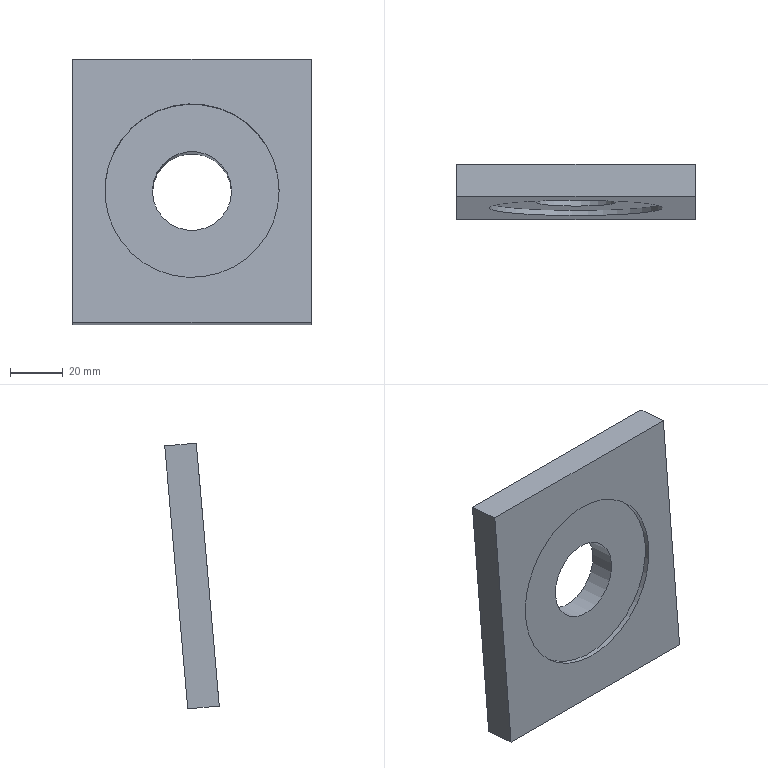Component | NX | REAR_BAFFLE | 1 solid | 9 faces | box 90.28 x 20.67 x 100.67 mm | volume 94428 mm3 | plane 7 | cylinder 2 | commonest cylinder face diameters 66 x1 30 x1
STEP:
#1=CARTESIAN_POINT('',(0.,0.,0.));
#2=DIRECTION('',(0.,0.,1.));
#3=DIRECTION('',(1.,0.,0.));
#4=AXIS2_PLACEMENT_3D('',#1,#2,#3);
#5=CARTESIAN_POINT('',(289.602,430.813,-47.513));
#6=VERTEX_POINT('',#5);
#7=CARTESIAN_POINT('',(379.884,430.813,-47.513));
#8=VERTEX_POINT('',#7);
#9=CARTESIAN_POINT('',(269.743,430.813,-47.513));
#10=DIRECTION('',(1.,0.,0.));
#11=VECTOR('',#10,1.);
#12=LINE('',#9,#11);
#13=CARTESIAN_POINT('',(269.743,418.858,-46.467));
#14=DIRECTION('',(0.,0.08716,0.9962));
#15=DIRECTION('',(0.,-0.9962,0.08716));
#16=AXIS2_PLACEMENT_3D('',#13,#14,#15);
#17=PLANE('',#16);
#18=CARTESIAN_POINT('',(-12.,0.));
#19=DIRECTION('',(0.,1.));
#20=VECTOR('',#19,1.);
#21=LINE('',#18,#20);
#22=(GEOMETRIC_REPRESENTATION_CONTEXT(2)PARAMETRIC_REPRESENTATION_CONTEXT()REPRESENTATION_CONTEXT('',''));
#23=DEFINITIONAL_REPRESENTATION('',(#21),#22);
#24=PCURVE('',#17,#23);
#25=CARTESIAN_POINT('',(334.743,435.17,2.297));
#26=DIRECTION('',(0.,-0.9962,0.08716));
#27=DIRECTION('',(1.,0.,0.));
#28=AXIS2_PLACEMENT_3D('',#25,#26,#27);
#29=PLANE('',#28);
#30=CARTESIAN_POINT('',(-65.,-50.));
#31=DIRECTION('',(1.,0.));
#32=VECTOR('',#31,1.);
#33=LINE('',#30,#32);
#34=(GEOMETRIC_REPRESENTATION_CONTEXT(2)PARAMETRIC_REPRESENTATION_CONTEXT()REPRESENTATION_CONTEXT('',''));
#35=DEFINITIONAL_REPRESENTATION('',(#33),#34);
#36=PCURVE('',#29,#35);
#37=SURFACE_CURVE('',#12,(#24,#36),.PCURVE_S1.);
#38=EDGE_CURVE('',#6,#8,#37,.T.);
#39=ORIENTED_EDGE('',*,*,#38,.T.);
#40=CARTESIAN_POINT('',(379.884,418.858,-46.467));
#41=VERTEX_POINT('',#40);
#42=CARTESIAN_POINT('',(379.884,498.554,-53.439));
#43=DIRECTION('',(0.,-0.9962,0.08716));
#44=VECTOR('',#43,1.);
#45=LINE('',#42,#44);
#46=CARTESIAN_POINT('',(-80.,110.141));
#47=DIRECTION('',(1.,0.));
#48=VECTOR('',#47,1.);
#49=LINE('',#46,#48);
#50=(GEOMETRIC_REPRESENTATION_CONTEXT(2)PARAMETRIC_REPRESENTATION_CONTEXT()REPRESENTATION_CONTEXT('',''));
#51=DEFINITIONAL_REPRESENTATION('',(#49),#50);
#52=PCURVE('',#17,#51);
#53=CARTESIAN_POINT('',(379.884,507.269,46.18));
#54=DIRECTION('',(-1.,0.,0.));
#55=DIRECTION('',(-0.,-0.08716,-0.9962));
#56=AXIS2_PLACEMENT_3D('',#53,#54,#55);
#57=PLANE('',#56);
#58=CARTESIAN_POINT('',(100.,-0.));
#59=DIRECTION('',(-0.,1.));
#60=VECTOR('',#59,1.);
#61=LINE('',#58,#60);
#62=(GEOMETRIC_REPRESENTATION_CONTEXT(2)PARAMETRIC_REPRESENTATION_CONTEXT()REPRESENTATION_CONTEXT('',''));
#63=DEFINITIONAL_REPRESENTATION('',(#61),#62);
#64=PCURVE('',#57,#63);
#65=SURFACE_CURVE('',#45,(#52,#64),.PCURVE_S1.);
#66=EDGE_CURVE('',#8,#41,#65,.T.);
#67=ORIENTED_EDGE('',*,*,#66,.T.);
#68=CARTESIAN_POINT('',(289.602,418.858,-46.467));
#69=VERTEX_POINT('',#68);
#70=CARTESIAN_POINT('',(269.743,418.858,-46.467));
#71=DIRECTION('',(1.,0.,0.));
#72=VECTOR('',#71,1.);
#73=LINE('',#70,#72);
#74=CARTESIAN_POINT('',(0.,0.));
#75=DIRECTION('',(0.,1.));
#76=VECTOR('',#75,1.);
#77=LINE('',#74,#76);
#78=(GEOMETRIC_REPRESENTATION_CONTEXT(2)PARAMETRIC_REPRESENTATION_CONTEXT()REPRESENTATION_CONTEXT('',''));
#79=DEFINITIONAL_REPRESENTATION('',(#77),#78);
#80=PCURVE('',#17,#79);
#81=CARTESIAN_POINT('',(334.743,423.216,3.343));
#82=DIRECTION('',(0.,-0.9962,0.08716));
#83=DIRECTION('',(1.,0.,0.));
#84=AXIS2_PLACEMENT_3D('',#81,#82,#83);
#85=PLANE('',#84);
#86=CARTESIAN_POINT('',(-65.,-50.));
#87=DIRECTION('',(1.,0.));
#88=VECTOR('',#87,1.);
#89=LINE('',#86,#88);
#90=(GEOMETRIC_REPRESENTATION_CONTEXT(2)PARAMETRIC_REPRESENTATION_CONTEXT()REPRESENTATION_CONTEXT('',''));
#91=DEFINITIONAL_REPRESENTATION('',(#89),#90);
#92=PCURVE('',#85,#91);
#93=SURFACE_CURVE('',#73,(#80,#92),.PCURVE_S1.);
#94=EDGE_CURVE('',#69,#41,#93,.T.);
#95=ORIENTED_EDGE('',*,*,#94,.F.);
#96=CARTESIAN_POINT('',(289.602,498.554,-53.439));
#97=DIRECTION('',(0.,-0.9962,0.08716));
#98=VECTOR('',#97,1.);
#99=LINE('',#96,#98);
#100=CARTESIAN_POINT('',(-80.,19.859));
#101=DIRECTION('',(1.,0.));
#102=VECTOR('',#101,1.);
#103=LINE('',#100,#102);
#104=(GEOMETRIC_REPRESENTATION_CONTEXT(2)PARAMETRIC_REPRESENTATION_CONTEXT()REPRESENTATION_CONTEXT('',''));
#105=DEFINITIONAL_REPRESENTATION('',(#103),#104);
#106=PCURVE('',#17,#105);
#107=CARTESIAN_POINT('',(289.602,498.554,-53.439));
#108=DIRECTION('',(1.,0.,0.));
#109=DIRECTION('',(0.,0.9962,-0.08716));
#110=AXIS2_PLACEMENT_3D('',#107,#108,#109);
#111=PLANE('',#110);
#112=CARTESIAN_POINT('',(0.,0.));
#113=DIRECTION('',(-1.,-0.));
#114=VECTOR('',#113,1.);
#115=LINE('',#112,#114);
#116=(GEOMETRIC_REPRESENTATION_CONTEXT(2)PARAMETRIC_REPRESENTATION_CONTEXT()REPRESENTATION_CONTEXT('',''));
#117=DEFINITIONAL_REPRESENTATION('',(#115),#116);
#118=PCURVE('',#111,#117);
#119=SURFACE_CURVE('',#99,(#106,#118),.PCURVE_S1.);
#120=EDGE_CURVE('',#6,#69,#119,.T.);
#121=ORIENTED_EDGE('',*,*,#120,.F.);
#122=EDGE_LOOP('',(#39,#67,#95,#121));
#123=FACE_BOUND('',#122,.T.);
#124=ADVANCED_FACE('',(#123),#17,.F.);
#125=CARTESIAN_POINT('',(379.884,439.528,52.107));
#126=VERTEX_POINT('',#125);
#127=CARTESIAN_POINT('',(379.884,427.574,53.153));
#128=VERTEX_POINT('',#127);
#129=CARTESIAN_POINT('',(379.884,507.269,46.18));
#130=DIRECTION('',(0.,-0.9962,0.08716));
#131=VECTOR('',#130,1.);
#132=LINE('',#129,#131);
#133=CARTESIAN_POINT('',(399.743,427.574,53.153));
#134=DIRECTION('',(0.,-0.08716,-0.9962));
#135=DIRECTION('',(0.,0.9962,-0.08716));
#136=AXIS2_PLACEMENT_3D('',#133,#134,#135);
#137=PLANE('',#136);
#138=CARTESIAN_POINT('',(80.,-19.859));
#139=DIRECTION('',(-1.,0.));
#140=VECTOR('',#139,1.);
#141=LINE('',#138,#140);
#142=(GEOMETRIC_REPRESENTATION_CONTEXT(2)PARAMETRIC_REPRESENTATION_CONTEXT()REPRESENTATION_CONTEXT('',''));
#143=DEFINITIONAL_REPRESENTATION('',(#141),#142);
#144=PCURVE('',#137,#143);
#145=CARTESIAN_POINT('',(0.,0.));
#146=DIRECTION('',(-0.,1.));
#147=VECTOR('',#146,1.);
#148=LINE('',#145,#147);
#149=(GEOMETRIC_REPRESENTATION_CONTEXT(2)PARAMETRIC_REPRESENTATION_CONTEXT()REPRESENTATION_CONTEXT('',''));
#150=DEFINITIONAL_REPRESENTATION('',(#148),#149);
#151=PCURVE('',#57,#150);
#152=SURFACE_CURVE('',#132,(#144,#151),.PCURVE_S1.);
#153=EDGE_CURVE('',#126,#128,#152,.T.);
#154=ORIENTED_EDGE('',*,*,#153,.F.);
#155=CARTESIAN_POINT('',(289.602,439.528,52.107));
#156=VERTEX_POINT('',#155);
#157=CARTESIAN_POINT('',(399.743,439.528,52.107));
#158=DIRECTION('',(-1.,0.,0.));
#159=VECTOR('',#158,1.);
#160=LINE('',#157,#159);
#161=CARTESIAN_POINT('',(12.,0.));
#162=DIRECTION('',(0.,-1.));
#163=VECTOR('',#162,1.);
#164=LINE('',#161,#163);
#165=(GEOMETRIC_REPRESENTATION_CONTEXT(2)PARAMETRIC_REPRESENTATION_CONTEXT()REPRESENTATION_CONTEXT('',''));
#166=DEFINITIONAL_REPRESENTATION('',(#164),#165);
#167=PCURVE('',#137,#166);
#168=CARTESIAN_POINT('',(65.,50.));
#169=DIRECTION('',(-1.,0.));
#170=VECTOR('',#169,1.);
#171=LINE('',#168,#170);
#172=(GEOMETRIC_REPRESENTATION_CONTEXT(2)PARAMETRIC_REPRESENTATION_CONTEXT()REPRESENTATION_CONTEXT('',''));
#173=DEFINITIONAL_REPRESENTATION('',(#171),#172);
#174=PCURVE('',#29,#173);
#175=SURFACE_CURVE('',#160,(#167,#174),.PCURVE_S1.);
#176=EDGE_CURVE('',#126,#156,#175,.T.);
#177=ORIENTED_EDGE('',*,*,#176,.T.);
#178=CARTESIAN_POINT('',(289.602,427.574,53.153));
#179=VERTEX_POINT('',#178);
#180=CARTESIAN_POINT('',(289.602,507.269,46.18));
#181=DIRECTION('',(0.,-0.9962,0.08716));
#182=VECTOR('',#181,1.);
#183=LINE('',#180,#182);
#184=CARTESIAN_POINT('',(80.,-110.141));
#185=DIRECTION('',(-1.,0.));
#186=VECTOR('',#185,1.);
#187=LINE('',#184,#186);
#188=(GEOMETRIC_REPRESENTATION_CONTEXT(2)PARAMETRIC_REPRESENTATION_CONTEXT()REPRESENTATION_CONTEXT('',''));
#189=DEFINITIONAL_REPRESENTATION('',(#187),#188);
#190=PCURVE('',#137,#189);
#191=CARTESIAN_POINT('',(-0.,100.));
#192=DIRECTION('',(-1.,-0.));
#193=VECTOR('',#192,1.);
#194=LINE('',#191,#193);
#195=(GEOMETRIC_REPRESENTATION_CONTEXT(2)PARAMETRIC_REPRESENTATION_CONTEXT()REPRESENTATION_CONTEXT('',''));
#196=DEFINITIONAL_REPRESENTATION('',(#194),#195);
#197=PCURVE('',#111,#196);
#198=SURFACE_CURVE('',#183,(#190,#197),.PCURVE_S1.);
#199=EDGE_CURVE('',#156,#179,#198,.T.);
#200=ORIENTED_EDGE('',*,*,#199,.T.);
#201=CARTESIAN_POINT('',(399.743,427.574,53.153));
#202=DIRECTION('',(-1.,0.,0.));
#203=VECTOR('',#202,1.);
#204=LINE('',#201,#203);
#205=CARTESIAN_POINT('',(0.,0.));
#206=DIRECTION('',(0.,-1.));
#207=VECTOR('',#206,1.);
#208=LINE('',#205,#207);
#209=(GEOMETRIC_REPRESENTATION_CONTEXT(2)PARAMETRIC_REPRESENTATION_CONTEXT()REPRESENTATION_CONTEXT('',''));
#210=DEFINITIONAL_REPRESENTATION('',(#208),#209);
#211=PCURVE('',#137,#210);
#212=CARTESIAN_POINT('',(65.,50.));
#213=DIRECTION('',(-1.,0.));
#214=VECTOR('',#213,1.);
#215=LINE('',#212,#214);
#216=(GEOMETRIC_REPRESENTATION_CONTEXT(2)PARAMETRIC_REPRESENTATION_CONTEXT()REPRESENTATION_CONTEXT('',''));
#217=DEFINITIONAL_REPRESENTATION('',(#215),#216);
#218=PCURVE('',#85,#217);
#219=SURFACE_CURVE('',#204,(#211,#218),.PCURVE_S1.);
#220=EDGE_CURVE('',#128,#179,#219,.T.);
#221=ORIENTED_EDGE('',*,*,#220,.F.);
#222=EDGE_LOOP('',(#154,#177,#200,#221));
#223=FACE_BOUND('',#222,.T.);
#224=ADVANCED_FACE('',(#223),#137,.F.);
#225=CARTESIAN_POINT('',(379.884,427.574,53.153));
#226=DIRECTION('',(-0.,-0.08716,-0.9962));
#227=VECTOR('',#226,1.);
#228=LINE('',#225,#227);
#229=CARTESIAN_POINT('',(45.141,50.));
#230=DIRECTION('',(-0.,-1.));
#231=VECTOR('',#230,1.);
#232=LINE('',#229,#231);
#233=(GEOMETRIC_REPRESENTATION_CONTEXT(2)PARAMETRIC_REPRESENTATION_CONTEXT()REPRESENTATION_CONTEXT('',''));
#234=DEFINITIONAL_REPRESENTATION('',(#232),#233);
#235=PCURVE('',#85,#234);
#236=CARTESIAN_POINT('',(-0.,80.));
#237=DIRECTION('',(1.,0.));
#238=VECTOR('',#237,1.);
#239=LINE('',#236,#238);
#240=(GEOMETRIC_REPRESENTATION_CONTEXT(2)PARAMETRIC_REPRESENTATION_CONTEXT()REPRESENTATION_CONTEXT('',''));
#241=DEFINITIONAL_REPRESENTATION('',(#239),#240);
#242=PCURVE('',#57,#241);
#243=SURFACE_CURVE('',#228,(#235,#242),.PCURVE_S1.);
#244=EDGE_CURVE('',#128,#41,#243,.T.);
#245=ORIENTED_EDGE('',*,*,#244,.F.);
#246=ORIENTED_EDGE('',*,*,#220,.T.);
#247=CARTESIAN_POINT('',(289.602,418.858,-46.467));
#248=DIRECTION('',(0.,0.08716,0.9962));
#249=VECTOR('',#248,1.);
#250=LINE('',#247,#249);
#251=CARTESIAN_POINT('',(-45.141,-50.));
#252=DIRECTION('',(0.,1.));
#253=VECTOR('',#252,1.);
#254=LINE('',#251,#253);
#255=(GEOMETRIC_REPRESENTATION_CONTEXT(2)PARAMETRIC_REPRESENTATION_CONTEXT()REPRESENTATION_CONTEXT('',''));
#256=DEFINITIONAL_REPRESENTATION('',(#254),#255);
#257=PCURVE('',#85,#256);
#258=CARTESIAN_POINT('',(-80.,-0.));
#259=DIRECTION('',(-0.,1.));
#260=VECTOR('',#259,1.);
#261=LINE('',#258,#260);
#262=(GEOMETRIC_REPRESENTATION_CONTEXT(2)PARAMETRIC_REPRESENTATION_CONTEXT()REPRESENTATION_CONTEXT('',''));
#263=DEFINITIONAL_REPRESENTATION('',(#261),#262);
#264=PCURVE('',#111,#263);
#265=SURFACE_CURVE('',#250,(#257,#264),.PCURVE_S1.);
#266=EDGE_CURVE('',#69,#179,#265,.T.);
#267=ORIENTED_EDGE('',*,*,#266,.F.);
#268=ORIENTED_EDGE('',*,*,#94,.T.);
#269=EDGE_LOOP('',(#245,#246,#267,#268));
#270=FACE_BOUND('',#269,.T.);
#271=CARTESIAN_POINT('',(367.743,423.216,3.343));
#272=VERTEX_POINT('',#271);
#273=CARTESIAN_POINT('',(334.743,423.216,3.343));
#274=DIRECTION('',(0.,-0.9962,0.08716));
#275=DIRECTION('',(1.,0.,0.));
#276=AXIS2_PLACEMENT_3D('',#273,#274,#275);
#277=CIRCLE('',#276,33.);
#278=CARTESIAN_POINT('',(0.,-0.));
#279=DIRECTION('',(1.,0.));
#280=AXIS2_PLACEMENT_2D('',#278,#279);
#281=CIRCLE('',#280,33.);
#282=(GEOMETRIC_REPRESENTATION_CONTEXT(2)PARAMETRIC_REPRESENTATION_CONTEXT()REPRESENTATION_CONTEXT('',''));
#283=DEFINITIONAL_REPRESENTATION('',(#281),#282);
#284=PCURVE('',#85,#283);
#285=CARTESIAN_POINT('',(334.743,425.208,3.169));
#286=DIRECTION('',(0.,-0.9962,0.08716));
#287=DIRECTION('',(1.,0.,0.));
#288=AXIS2_PLACEMENT_3D('',#285,#286,#287);
#289=CYLINDRICAL_SURFACE('',#288,33.);
#290=CARTESIAN_POINT('',(0.,2.));
#291=DIRECTION('',(1.,0.));
#292=VECTOR('',#291,1.);
#293=LINE('',#290,#292);
#294=(GEOMETRIC_REPRESENTATION_CONTEXT(2)PARAMETRIC_REPRESENTATION_CONTEXT()REPRESENTATION_CONTEXT('',''));
#295=DEFINITIONAL_REPRESENTATION('',(#293),#294);
#296=PCURVE('',#289,#295);
#297=SURFACE_CURVE('',#277,(#284,#296),.PCURVE_S1.);
#298=EDGE_CURVE('',#272,#272,#297,.T.);
#299=ORIENTED_EDGE('',*,*,#298,.F.);
#300=EDGE_LOOP('',(#299));
#301=FACE_BOUND('',#300,.T.);
#302=ADVANCED_FACE('',(#270,#301),#85,.T.);
#303=CARTESIAN_POINT('',(349.743,435.17,2.297));
#304=VERTEX_POINT('',#303);
#305=CARTESIAN_POINT('',(334.743,435.17,2.297));
#306=DIRECTION('',(0.,-0.9962,0.08716));
#307=DIRECTION('',(1.,0.,0.));
#308=AXIS2_PLACEMENT_3D('',#305,#306,#307);
#309=CIRCLE('',#308,15.);
#310=CARTESIAN_POINT('',(0.,0.));
#311=DIRECTION('',(1.,0.));
#312=AXIS2_PLACEMENT_2D('',#310,#311);
#313=CIRCLE('',#312,15.);
#314=(GEOMETRIC_REPRESENTATION_CONTEXT(2)PARAMETRIC_REPRESENTATION_CONTEXT()REPRESENTATION_CONTEXT('',''));
#315=DEFINITIONAL_REPRESENTATION('',(#313),#314);
#316=PCURVE('',#29,#315);
#317=CARTESIAN_POINT('',(334.743,476.014,-1.276));
#318=DIRECTION('',(0.,-0.9962,0.08716));
#319=DIRECTION('',(1.,0.,0.));
#320=AXIS2_PLACEMENT_3D('',#317,#318,#319);
#321=CYLINDRICAL_SURFACE('',#320,15.);
#322=CARTESIAN_POINT('',(0.,41.));
#323=DIRECTION('',(1.,0.));
#324=VECTOR('',#323,1.);
#325=LINE('',#322,#324);
#326=(GEOMETRIC_REPRESENTATION_CONTEXT(2)PARAMETRIC_REPRESENTATION_CONTEXT()REPRESENTATION_CONTEXT('',''));
#327=DEFINITIONAL_REPRESENTATION('',(#325),#326);
#328=PCURVE('',#321,#327);
#329=SURFACE_CURVE('',#309,(#316,#328),.PCURVE_S1.);
#330=EDGE_CURVE('',#304,#304,#329,.T.);
#331=ORIENTED_EDGE('',*,*,#330,.T.);
#332=EDGE_LOOP('',(#331));
#333=FACE_BOUND('',#332,.T.);
#334=ORIENTED_EDGE('',*,*,#176,.F.);
#335=CARTESIAN_POINT('',(379.884,435.17,2.297));
#336=DIRECTION('',(-0.,-0.08716,-0.9962));
#337=VECTOR('',#336,1.);
#338=LINE('',#335,#337);
#339=CARTESIAN_POINT('',(45.141,-0.));
#340=DIRECTION('',(-0.,-1.));
#341=VECTOR('',#340,1.);
#342=LINE('',#339,#341);
#343=(GEOMETRIC_REPRESENTATION_CONTEXT(2)PARAMETRIC_REPRESENTATION_CONTEXT()REPRESENTATION_CONTEXT('',''));
#344=DEFINITIONAL_REPRESENTATION('',(#342),#343);
#345=PCURVE('',#29,#344);
#346=CARTESIAN_POINT('',(50.,68.));
#347=DIRECTION('',(1.,0.));
#348=VECTOR('',#347,1.);
#349=LINE('',#346,#348);
#350=(GEOMETRIC_REPRESENTATION_CONTEXT(2)PARAMETRIC_REPRESENTATION_CONTEXT()REPRESENTATION_CONTEXT('',''));
#351=DEFINITIONAL_REPRESENTATION('',(#349),#350);
#352=PCURVE('',#57,#351);
#353=SURFACE_CURVE('',#338,(#345,#352),.PCURVE_S1.);
#354=EDGE_CURVE('',#126,#8,#353,.T.);
#355=ORIENTED_EDGE('',*,*,#354,.T.);
#356=ORIENTED_EDGE('',*,*,#38,.F.);
#357=CARTESIAN_POINT('',(289.602,435.17,2.297));
#358=DIRECTION('',(0.,0.08716,0.9962));
#359=VECTOR('',#358,1.);
#360=LINE('',#357,#359);
#361=CARTESIAN_POINT('',(-45.141,0.));
#362=DIRECTION('',(0.,1.));
#363=VECTOR('',#362,1.);
#364=LINE('',#361,#363);
#365=(GEOMETRIC_REPRESENTATION_CONTEXT(2)PARAMETRIC_REPRESENTATION_CONTEXT()REPRESENTATION_CONTEXT('',''));
#366=DEFINITIONAL_REPRESENTATION('',(#364),#365);
#367=PCURVE('',#29,#366);
#368=CARTESIAN_POINT('',(-68.,50.));
#369=DIRECTION('',(-0.,1.));
#370=VECTOR('',#369,1.);
#371=LINE('',#368,#370);
#372=(GEOMETRIC_REPRESENTATION_CONTEXT(2)PARAMETRIC_REPRESENTATION_CONTEXT()REPRESENTATION_CONTEXT('',''));
#373=DEFINITIONAL_REPRESENTATION('',(#371),#372);
#374=PCURVE('',#111,#373);
#375=SURFACE_CURVE('',#360,(#367,#374),.PCURVE_S1.);
#376=EDGE_CURVE('',#6,#156,#375,.T.);
#377=ORIENTED_EDGE('',*,*,#376,.T.);
#378=EDGE_LOOP('',(#334,#355,#356,#377));
#379=FACE_BOUND('',#378,.T.);
#380=ADVANCED_FACE('',(#333,#379),#29,.F.);
#381=CARTESIAN_POINT('',(367.743,425.208,3.169));
#382=VERTEX_POINT('',#381);
#383=CARTESIAN_POINT('',(334.743,425.208,3.169));
#384=DIRECTION('',(0.,0.9962,-0.08716));
#385=DIRECTION('',(1.,0.,0.));
#386=AXIS2_PLACEMENT_3D('',#383,#384,#385);
#387=CIRCLE('',#386,33.);
#388=CARTESIAN_POINT('',(6.283,0.));
#389=DIRECTION('',(-1.,0.));
#390=VECTOR('',#389,1.);
#391=LINE('',#388,#390);
#392=(GEOMETRIC_REPRESENTATION_CONTEXT(2)PARAMETRIC_REPRESENTATION_CONTEXT()REPRESENTATION_CONTEXT('',''));
#393=DEFINITIONAL_REPRESENTATION('',(#391),#392);
#394=PCURVE('',#289,#393);
#395=CARTESIAN_POINT('',(334.743,425.208,3.169));
#396=DIRECTION('',(0.,-0.9962,0.08716));
#397=DIRECTION('',(1.,0.,0.));
#398=AXIS2_PLACEMENT_3D('',#395,#396,#397);
#399=PLANE('',#398);
#400=CARTESIAN_POINT('',(33.,0.));
#401=CARTESIAN_POINT('',(33.,-57.158));
#402=CARTESIAN_POINT('',(-16.5,-28.579));
#403=CARTESIAN_POINT('',(-66.,-0.));
#404=CARTESIAN_POINT('',(-16.5,28.579));
#405=CARTESIAN_POINT('',(33.,57.158));
#406=CARTESIAN_POINT('',(33.,0.));
#407=(BOUNDED_CURVE()B_SPLINE_CURVE(2,(#400,#401,#402,#403,#404,#405,#406),.UNSPECIFIED.,.T.,.F.)B_SPLINE_CURVE_WITH_KNOTS((1,2,2,2,2,1),(-2.094,0.,2.094,4.189,6.283,8.378),.UNSPECIFIED.)CURVE()GEOMETRIC_REPRESENTATION_ITEM()RATIONAL_B_SPLINE_CURVE((1.,0.5,1.,0.5,1.,0.5,1.))REPRESENTATION_ITEM(''));
#408=(GEOMETRIC_REPRESENTATION_CONTEXT(2)PARAMETRIC_REPRESENTATION_CONTEXT()REPRESENTATION_CONTEXT('',''));
#409=DEFINITIONAL_REPRESENTATION('',(#407),#408);
#410=PCURVE('',#399,#409);
#411=SURFACE_CURVE('',#387,(#394,#410),.PCURVE_S1.);
#412=EDGE_CURVE('',#382,#382,#411,.T.);
#413=ORIENTED_EDGE('',*,*,#412,.F.);
#414=CARTESIAN_POINT('',(367.743,425.208,3.169));
#415=CARTESIAN_POINT('',(367.743,423.216,3.343));
#416=B_SPLINE_CURVE_WITH_KNOTS('',1,(#414,#415),.UNSPECIFIED.,.F.,.F.,(2,2),(0.,2.),.PIECEWISE_BEZIER_KNOTS.);
#417=CARTESIAN_POINT('',(6.283,0.));
#418=DIRECTION('',(0.,1.));
#419=VECTOR('',#418,1.);
#420=LINE('',#417,#419);
#421=(GEOMETRIC_REPRESENTATION_CONTEXT(2)PARAMETRIC_REPRESENTATION_CONTEXT()REPRESENTATION_CONTEXT('',''));
#422=DEFINITIONAL_REPRESENTATION('',(#420),#421);
#423=PCURVE('',#289,#422);
#424=CARTESIAN_POINT('',(0.,0.));
#425=DIRECTION('',(0.,1.));
#426=VECTOR('',#425,1.);
#427=LINE('',#424,#426);
#428=(GEOMETRIC_REPRESENTATION_CONTEXT(2)PARAMETRIC_REPRESENTATION_CONTEXT()REPRESENTATION_CONTEXT('',''));
#429=DEFINITIONAL_REPRESENTATION('',(#427),#428);
#430=PCURVE('',#289,#429);
#431=SEAM_CURVE('',#416,(#423,#430),.PCURVE_S1.);
#432=EDGE_CURVE('',#382,#272,#431,.T.);
#433=ORIENTED_EDGE('',*,*,#432,.T.);
#434=ORIENTED_EDGE('',*,*,#298,.F.);
#435=ORIENTED_EDGE('',*,*,#432,.F.);
#436=EDGE_LOOP('',(#413,#433,#434,#435));
#437=FACE_BOUND('',#436,.F.);
#438=ADVANCED_FACE('',(#437),#289,.F.);
#439=CARTESIAN_POINT('',(349.743,425.208,3.169));
#440=VERTEX_POINT('',#439);
#441=CARTESIAN_POINT('',(334.743,425.208,3.169));
#442=DIRECTION('',(0.,-0.9962,0.08716));
#443=DIRECTION('',(1.,0.,0.));
#444=AXIS2_PLACEMENT_3D('',#441,#442,#443);
#445=CIRCLE('',#444,15.);
#446=CARTESIAN_POINT('',(0.,0.));
#447=DIRECTION('',(1.,0.));
#448=AXIS2_PLACEMENT_2D('',#446,#447);
#449=CIRCLE('',#448,15.);
#450=(GEOMETRIC_REPRESENTATION_CONTEXT(2)PARAMETRIC_REPRESENTATION_CONTEXT()REPRESENTATION_CONTEXT('',''));
#451=DEFINITIONAL_REPRESENTATION('',(#449),#450);
#452=PCURVE('',#399,#451);
#453=CARTESIAN_POINT('',(0.,51.));
#454=DIRECTION('',(1.,0.));
#455=VECTOR('',#454,1.);
#456=LINE('',#453,#455);
#457=(GEOMETRIC_REPRESENTATION_CONTEXT(2)PARAMETRIC_REPRESENTATION_CONTEXT()REPRESENTATION_CONTEXT('',''));
#458=DEFINITIONAL_REPRESENTATION('',(#456),#457);
#459=PCURVE('',#321,#458);
#460=SURFACE_CURVE('',#445,(#452,#459),.PCURVE_S1.);
#461=EDGE_CURVE('',#440,#440,#460,.T.);
#462=ORIENTED_EDGE('',*,*,#461,.F.);
#463=EDGE_LOOP('',(#462));
#464=FACE_BOUND('',#463,.T.);
#465=ORIENTED_EDGE('',*,*,#412,.F.);
#466=EDGE_LOOP('',(#465));
#467=FACE_BOUND('',#466,.T.);
#468=ADVANCED_FACE('',(#464,#467),#399,.T.);
#469=ORIENTED_EDGE('',*,*,#461,.F.);
#470=CARTESIAN_POINT('',(349.743,435.17,2.297));
#471=CARTESIAN_POINT('',(349.743,425.208,3.169));
#472=B_SPLINE_CURVE_WITH_KNOTS('',1,(#470,#471),.UNSPECIFIED.,.F.,.F.,(2,2),(41.,51.),.PIECEWISE_BEZIER_KNOTS.);
#473=CARTESIAN_POINT('',(0.,0.));
#474=DIRECTION('',(0.,1.));
#475=VECTOR('',#474,1.);
#476=LINE('',#473,#475);
#477=(GEOMETRIC_REPRESENTATION_CONTEXT(2)PARAMETRIC_REPRESENTATION_CONTEXT()REPRESENTATION_CONTEXT('',''));
#478=DEFINITIONAL_REPRESENTATION('',(#476),#477);
#479=PCURVE('',#321,#478);
#480=CARTESIAN_POINT('',(6.283,0.));
#481=DIRECTION('',(0.,1.));
#482=VECTOR('',#481,1.);
#483=LINE('',#480,#482);
#484=(GEOMETRIC_REPRESENTATION_CONTEXT(2)PARAMETRIC_REPRESENTATION_CONTEXT()REPRESENTATION_CONTEXT('',''));
#485=DEFINITIONAL_REPRESENTATION('',(#483),#484);
#486=PCURVE('',#321,#485);
#487=SEAM_CURVE('',#472,(#479,#486),.PCURVE_S1.);
#488=EDGE_CURVE('',#304,#440,#487,.T.);
#489=ORIENTED_EDGE('',*,*,#488,.F.);
#490=ORIENTED_EDGE('',*,*,#330,.T.);
#491=ORIENTED_EDGE('',*,*,#488,.T.);
#492=EDGE_LOOP('',(#469,#489,#490,#491));
#493=FACE_BOUND('',#492,.F.);
#494=ADVANCED_FACE('',(#493),#321,.F.);
#495=ORIENTED_EDGE('',*,*,#120,.T.);
#496=ORIENTED_EDGE('',*,*,#266,.T.);
#497=ORIENTED_EDGE('',*,*,#199,.F.);
#498=ORIENTED_EDGE('',*,*,#376,.F.);
#499=EDGE_LOOP('',(#495,#496,#497,#498));
#500=FACE_BOUND('',#499,.T.);
#501=ADVANCED_FACE('',(#500),#111,.F.);
#502=ORIENTED_EDGE('',*,*,#153,.T.);
#503=ORIENTED_EDGE('',*,*,#244,.T.);
#504=ORIENTED_EDGE('',*,*,#66,.F.);
#505=ORIENTED_EDGE('',*,*,#354,.F.);
#506=EDGE_LOOP('',(#502,#503,#504,#505));
#507=FACE_BOUND('',#506,.T.);
#508=ADVANCED_FACE('',(#507),#57,.F.);
#509=CLOSED_SHELL('',(#124,#224,#302,#380,#438,#468,#494,#501,#508));
#510=MANIFOLD_SOLID_BREP('',#509);
#511=(LENGTH_UNIT()NAMED_UNIT(*)SI_UNIT(.MILLI.,.METRE.));
#512=UNCERTAINTY_MEASURE_WITH_UNIT(LENGTH_MEASURE(0.000002),#511,'','');
#513=(NAMED_UNIT(*)PLANE_ANGLE_UNIT()SI_UNIT($,.RADIAN.));
#514=(NAMED_UNIT(*)SI_UNIT($,.STERADIAN.)SOLID_ANGLE_UNIT());
#515=(GEOMETRIC_REPRESENTATION_CONTEXT(3)GLOBAL_UNCERTAINTY_ASSIGNED_CONTEXT((#512))GLOBAL_UNIT_ASSIGNED_CONTEXT((#511,#513,#514))REPRESENTATION_CONTEXT('',''));
#516=ADVANCED_BREP_SHAPE_REPRESENTATION('',(#4,#510),#515);